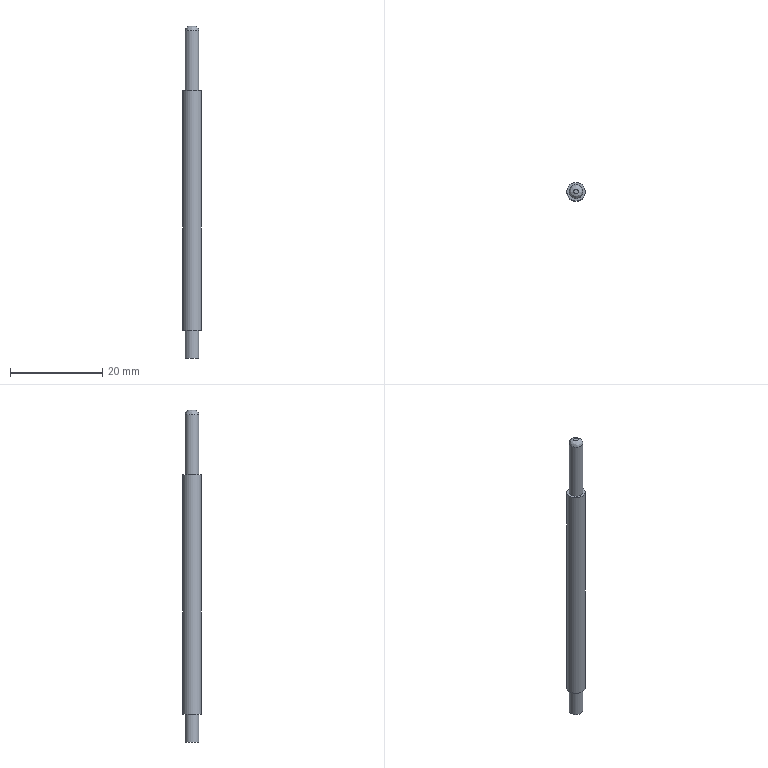Component | NX | CONN_SHAFT_1 | 1 solid | 8 faces | box 4 x 4 x 72 mm | volume 793 mm3 | plane 4 | cylinder 3 | spline 1 | commonest cylinder face diameters 3 x2 4 x1
STEP:
#1=CARTESIAN_POINT('',(0.,0.,0.));
#2=DIRECTION('',(0.,0.,1.));
#3=DIRECTION('',(1.,0.,0.));
#4=AXIS2_PLACEMENT_3D('',#1,#2,#3);
#5=CARTESIAN_POINT('',(0.004666,23.5,164.631));
#6=VERTEX_POINT('',#5);
#7=CARTESIAN_POINT('',(-0.,23.,164.631));
#8=DIRECTION('',(0.,0.,1.));
#9=DIRECTION('',(0.009333,1.,0.));
#10=AXIS2_PLACEMENT_3D('',#7,#8,#9);
#11=CIRCLE('',#10,0.5);
#12=CARTESIAN_POINT('',(-0.,23.,164.631));
#13=DIRECTION('',(0.,0.,1.));
#14=DIRECTION('',(0.009333,1.,0.));
#15=AXIS2_PLACEMENT_3D('',#12,#13,#14);
#16=PLANE('',#15);
#17=CARTESIAN_POINT('',(0.,0.));
#18=DIRECTION('',(1.,0.));
#19=AXIS2_PLACEMENT_2D('',#17,#18);
#20=CIRCLE('',#19,0.5);
#21=(GEOMETRIC_REPRESENTATION_CONTEXT(2)PARAMETRIC_REPRESENTATION_CONTEXT()REPRESENTATION_CONTEXT('',''));
#22=DEFINITIONAL_REPRESENTATION('',(#20),#21);
#23=PCURVE('',#16,#22);
#24=CARTESIAN_POINT('',(0.004666,23.5,164.631));
#25=CARTESIAN_POINT('',(-0.9953,23.509,164.631));
#26=CARTESIAN_POINT('',(-1.005,22.509,164.631));
#27=CARTESIAN_POINT('',(-0.004666,22.5,164.631));
#28=CARTESIAN_POINT('',(0.9953,22.491,164.631));
#29=CARTESIAN_POINT('',(1.005,23.491,164.631));
#30=CARTESIAN_POINT('',(0.004666,23.5,164.631));
#31=CARTESIAN_POINT('',(0.01013,24.086,164.631));
#32=CARTESIAN_POINT('',(-2.161,24.106,164.631));
#33=CARTESIAN_POINT('',(-2.182,21.935,164.631));
#34=CARTESIAN_POINT('',(-0.01013,21.914,164.631));
#35=CARTESIAN_POINT('',(2.161,21.894,164.631));
#36=CARTESIAN_POINT('',(2.182,24.065,164.631));
#37=CARTESIAN_POINT('',(0.01013,24.086,164.631));
#38=CARTESIAN_POINT('',(0.014,24.5,164.217));
#39=CARTESIAN_POINT('',(-2.986,24.528,164.217));
#40=CARTESIAN_POINT('',(-3.014,21.528,164.217));
#41=CARTESIAN_POINT('',(-0.014,21.5,164.217));
#42=CARTESIAN_POINT('',(2.986,21.472,164.217));
#43=CARTESIAN_POINT('',(3.014,24.472,164.217));
#44=CARTESIAN_POINT('',(0.014,24.5,164.217));
#45=CARTESIAN_POINT('',(0.014,24.5,163.631));
#46=CARTESIAN_POINT('',(-2.986,24.528,163.631));
#47=CARTESIAN_POINT('',(-3.014,21.528,163.631));
#48=CARTESIAN_POINT('',(-0.014,21.5,163.631));
#49=CARTESIAN_POINT('',(2.986,21.472,163.631));
#50=CARTESIAN_POINT('',(3.014,24.472,163.631));
#51=CARTESIAN_POINT('',(0.014,24.5,163.631));
#52=(BOUNDED_SURFACE()B_SPLINE_SURFACE(3,3,((#24,#25,#26,#27,#28,#29,#30),(#31,#32,#33,#34,#35,#36,#37),(#38,#39,#40,#41,#42,#43,#44),(#45,#46,#47,#48,#49,#50,#51)),.UNSPECIFIED.,.F.,.T.,.F.)B_SPLINE_SURFACE_WITH_KNOTS((4,4),(1,3,3,3,1),(0.,1.),(-0.5,0.,0.5,1.,1.5),.UNSPECIFIED.)GEOMETRIC_REPRESENTATION_ITEM()RATIONAL_B_SPLINE_SURFACE(((1.,0.3333,0.3333,1.,0.3333,0.3333,1.),(0.8047,0.2682,0.2682,0.8047,0.2682,0.2682,0.8047),(0.8047,0.2682,0.2682,0.8047,0.2682,0.2682,0.8047),(1.,0.3333,0.3333,1.,0.3333,0.3333,1.)))REPRESENTATION_ITEM('')SURFACE());
#53=CARTESIAN_POINT('',(0.,0.));
#54=CARTESIAN_POINT('',(0.,0.02352));
#55=CARTESIAN_POINT('',(0.,0.06491));
#56=CARTESIAN_POINT('',(0.,0.1146));
#57=CARTESIAN_POINT('',(0.,0.1575));
#58=CARTESIAN_POINT('',(0.,0.196));
#59=CARTESIAN_POINT('',(0.,0.2322));
#60=CARTESIAN_POINT('',(0.,0.2678));
#61=CARTESIAN_POINT('',(0.,0.304));
#62=CARTESIAN_POINT('',(0.,0.3425));
#63=CARTESIAN_POINT('',(0.,0.3856));
#64=CARTESIAN_POINT('',(0.,0.4343));
#65=CARTESIAN_POINT('',(0.,0.5));
#66=CARTESIAN_POINT('',(0.,0.5657));
#67=CARTESIAN_POINT('',(0.,0.6144));
#68=CARTESIAN_POINT('',(0.,0.6575));
#69=CARTESIAN_POINT('',(0.,0.696));
#70=CARTESIAN_POINT('',(0.,0.7322));
#71=CARTESIAN_POINT('',(0.,0.7678));
#72=CARTESIAN_POINT('',(0.,0.804));
#73=CARTESIAN_POINT('',(0.,0.8425));
#74=CARTESIAN_POINT('',(0.,0.8854));
#75=CARTESIAN_POINT('',(0.,0.9351));
#76=CARTESIAN_POINT('',(0.,0.9765));
#77=CARTESIAN_POINT('',(0.,1.));
#78=B_SPLINE_CURVE_WITH_KNOTS('',3,(#53,#54,#55,#56,#57,#58,#59,#60,#61,#62,#63,#64,#65,#66,#67,#68,#69,#70,#71,#72,#73,#74,#75,#76,#77),.UNSPECIFIED.,.F.,.F.,(4,1,1,1,1,1,1,1,1,1,1,1,1,1,1,1,1,1,1,1,1,1,4),(0.,0.2856,0.5712,0.8568,1.142,1.428,1.714,1.999,2.285,2.57,2.856,3.142,3.427,3.713,3.998,4.284,4.57,4.855,5.141,5.426,5.712,5.998,6.283),.QUASI_UNIFORM_KNOTS.);
#79=(GEOMETRIC_REPRESENTATION_CONTEXT(2)PARAMETRIC_REPRESENTATION_CONTEXT()REPRESENTATION_CONTEXT('',''));
#80=DEFINITIONAL_REPRESENTATION('',(#78),#79);
#81=PCURVE('',#52,#80);
#82=SURFACE_CURVE('',#11,(#23,#81),.PCURVE_S1.);
#83=EDGE_CURVE('',#6,#6,#82,.T.);
#84=ORIENTED_EDGE('',*,*,#83,.T.);
#85=EDGE_LOOP('',(#84));
#86=FACE_BOUND('',#85,.T.);
#87=ADVANCED_FACE('',(#86),#16,.T.);
#88=CARTESIAN_POINT('',(0.014,24.5,163.631));
#89=VERTEX_POINT('',#88);
#90=CARTESIAN_POINT('',(-0.,23.,163.631));
#91=DIRECTION('',(0.,0.,-1.));
#92=DIRECTION('',(0.009333,1.,0.));
#93=AXIS2_PLACEMENT_3D('',#90,#91,#92);
#94=CIRCLE('',#93,1.5);
#95=CARTESIAN_POINT('',(-0.,23.,150.631));
#96=DIRECTION('',(0.,0.,1.));
#97=DIRECTION('',(0.009333,1.,0.));
#98=AXIS2_PLACEMENT_3D('',#95,#96,#97);
#99=CYLINDRICAL_SURFACE('',#98,1.5);
#100=CARTESIAN_POINT('',(6.283,13.));
#101=DIRECTION('',(-1.,0.));
#102=VECTOR('',#101,1.);
#103=LINE('',#100,#102);
#104=(GEOMETRIC_REPRESENTATION_CONTEXT(2)PARAMETRIC_REPRESENTATION_CONTEXT()REPRESENTATION_CONTEXT('',''));
#105=DEFINITIONAL_REPRESENTATION('',(#103),#104);
#106=PCURVE('',#99,#105);
#107=CARTESIAN_POINT('',(1.,1.));
#108=CARTESIAN_POINT('',(1.,0.9765));
#109=CARTESIAN_POINT('',(1.,0.9351));
#110=CARTESIAN_POINT('',(1.,0.8854));
#111=CARTESIAN_POINT('',(1.,0.8425));
#112=CARTESIAN_POINT('',(1.,0.804));
#113=CARTESIAN_POINT('',(1.,0.7678));
#114=CARTESIAN_POINT('',(1.,0.7322));
#115=CARTESIAN_POINT('',(1.,0.696));
#116=CARTESIAN_POINT('',(1.,0.6575));
#117=CARTESIAN_POINT('',(1.,0.6144));
#118=CARTESIAN_POINT('',(1.,0.5657));
#119=CARTESIAN_POINT('',(1.,0.5));
#120=CARTESIAN_POINT('',(1.,0.4343));
#121=CARTESIAN_POINT('',(1.,0.3856));
#122=CARTESIAN_POINT('',(1.,0.3425));
#123=CARTESIAN_POINT('',(1.,0.304));
#124=CARTESIAN_POINT('',(1.,0.2678));
#125=CARTESIAN_POINT('',(1.,0.2322));
#126=CARTESIAN_POINT('',(1.,0.196));
#127=CARTESIAN_POINT('',(1.,0.1575));
#128=CARTESIAN_POINT('',(1.,0.1146));
#129=CARTESIAN_POINT('',(1.,0.06491));
#130=CARTESIAN_POINT('',(1.,0.02352));
#131=CARTESIAN_POINT('',(1.,0.));
#132=B_SPLINE_CURVE_WITH_KNOTS('',3,(#107,#108,#109,#110,#111,#112,#113,#114,#115,#116,#117,#118,#119,#120,#121,#122,#123,#124,#125,#126,#127,#128,#129,#130,#131),.UNSPECIFIED.,.F.,.F.,(4,1,1,1,1,1,1,1,1,1,1,1,1,1,1,1,1,1,1,1,1,1,4),(0.,0.2856,0.5712,0.8568,1.142,1.428,1.714,1.999,2.285,2.57,2.856,3.142,3.427,3.713,3.998,4.284,4.57,4.855,5.141,5.426,5.712,5.998,6.283),.QUASI_UNIFORM_KNOTS.);
#133=(GEOMETRIC_REPRESENTATION_CONTEXT(2)PARAMETRIC_REPRESENTATION_CONTEXT()REPRESENTATION_CONTEXT('',''));
#134=DEFINITIONAL_REPRESENTATION('',(#132),#133);
#135=PCURVE('',#52,#134);
#136=SURFACE_CURVE('',#94,(#106,#135),.PCURVE_S1.);
#137=EDGE_CURVE('',#89,#89,#136,.T.);
#138=ORIENTED_EDGE('',*,*,#137,.T.);
#139=CARTESIAN_POINT('',(0.014,24.5,150.631));
#140=VERTEX_POINT('',#139);
#141=CARTESIAN_POINT('',(0.014,24.5,150.631));
#142=CARTESIAN_POINT('',(0.014,24.5,163.631));
#143=B_SPLINE_CURVE_WITH_KNOTS('',1,(#141,#142),.UNSPECIFIED.,.F.,.F.,(2,2),(0.,13.),.PIECEWISE_BEZIER_KNOTS.);
#144=CARTESIAN_POINT('',(0.,0.));
#145=DIRECTION('',(0.,1.));
#146=VECTOR('',#145,1.);
#147=LINE('',#144,#146);
#148=(GEOMETRIC_REPRESENTATION_CONTEXT(2)PARAMETRIC_REPRESENTATION_CONTEXT()REPRESENTATION_CONTEXT('',''));
#149=DEFINITIONAL_REPRESENTATION('',(#147),#148);
#150=PCURVE('',#99,#149);
#151=CARTESIAN_POINT('',(6.283,0.));
#152=DIRECTION('',(0.,1.));
#153=VECTOR('',#152,1.);
#154=LINE('',#151,#153);
#155=(GEOMETRIC_REPRESENTATION_CONTEXT(2)PARAMETRIC_REPRESENTATION_CONTEXT()REPRESENTATION_CONTEXT('',''));
#156=DEFINITIONAL_REPRESENTATION('',(#154),#155);
#157=PCURVE('',#99,#156);
#158=SEAM_CURVE('',#143,(#150,#157),.PCURVE_S1.);
#159=EDGE_CURVE('',#140,#89,#158,.T.);
#160=ORIENTED_EDGE('',*,*,#159,.F.);
#161=CARTESIAN_POINT('',(-0.,23.,150.631));
#162=DIRECTION('',(0.,0.,1.));
#163=DIRECTION('',(0.009333,1.,0.));
#164=AXIS2_PLACEMENT_3D('',#161,#162,#163);
#165=CIRCLE('',#164,1.5);
#166=CARTESIAN_POINT('',(0.,0.));
#167=DIRECTION('',(1.,0.));
#168=VECTOR('',#167,1.);
#169=LINE('',#166,#168);
#170=(GEOMETRIC_REPRESENTATION_CONTEXT(2)PARAMETRIC_REPRESENTATION_CONTEXT()REPRESENTATION_CONTEXT('',''));
#171=DEFINITIONAL_REPRESENTATION('',(#169),#170);
#172=PCURVE('',#99,#171);
#173=CARTESIAN_POINT('',(-0.,23.,150.631));
#174=DIRECTION('',(0.,0.,1.));
#175=DIRECTION('',(0.009333,1.,0.));
#176=AXIS2_PLACEMENT_3D('',#173,#174,#175);
#177=PLANE('',#176);
#178=CARTESIAN_POINT('',(0.,-0.));
#179=DIRECTION('',(1.,0.));
#180=AXIS2_PLACEMENT_2D('',#178,#179);
#181=CIRCLE('',#180,1.5);
#182=(GEOMETRIC_REPRESENTATION_CONTEXT(2)PARAMETRIC_REPRESENTATION_CONTEXT()REPRESENTATION_CONTEXT('',''));
#183=DEFINITIONAL_REPRESENTATION('',(#181),#182);
#184=PCURVE('',#177,#183);
#185=SURFACE_CURVE('',#165,(#172,#184),.PCURVE_S1.);
#186=EDGE_CURVE('',#140,#140,#185,.T.);
#187=ORIENTED_EDGE('',*,*,#186,.T.);
#188=ORIENTED_EDGE('',*,*,#159,.T.);
#189=EDGE_LOOP('',(#138,#160,#187,#188));
#190=FACE_BOUND('',#189,.T.);
#191=ADVANCED_FACE('',(#190),#99,.T.);
#192=CARTESIAN_POINT('',(-0.014,21.5,98.631));
#193=VERTEX_POINT('',#192);
#194=CARTESIAN_POINT('',(-0.,23.,98.631));
#195=DIRECTION('',(0.,0.,-1.));
#196=DIRECTION('',(-0.009333,-1.,0.));
#197=AXIS2_PLACEMENT_3D('',#194,#195,#196);
#198=CIRCLE('',#197,1.5);
#199=CARTESIAN_POINT('',(-0.,23.,98.631));
#200=DIRECTION('',(0.,0.,-1.));
#201=DIRECTION('',(-0.009333,-1.,0.));
#202=AXIS2_PLACEMENT_3D('',#199,#200,#201);
#203=PLANE('',#202);
#204=CARTESIAN_POINT('',(-0.,-0.));
#205=DIRECTION('',(1.,0.));
#206=AXIS2_PLACEMENT_2D('',#204,#205);
#207=CIRCLE('',#206,1.5);
#208=(GEOMETRIC_REPRESENTATION_CONTEXT(2)PARAMETRIC_REPRESENTATION_CONTEXT()REPRESENTATION_CONTEXT('',''));
#209=DEFINITIONAL_REPRESENTATION('',(#207),#208);
#210=PCURVE('',#203,#209);
#211=CARTESIAN_POINT('',(-0.,23.,98.631));
#212=DIRECTION('',(0.,0.,-1.));
#213=DIRECTION('',(-0.009333,-1.,0.));
#214=AXIS2_PLACEMENT_3D('',#211,#212,#213);
#215=CYLINDRICAL_SURFACE('',#214,1.5);
#216=CARTESIAN_POINT('',(0.,0.));
#217=DIRECTION('',(1.,0.));
#218=VECTOR('',#217,1.);
#219=LINE('',#216,#218);
#220=(GEOMETRIC_REPRESENTATION_CONTEXT(2)PARAMETRIC_REPRESENTATION_CONTEXT()REPRESENTATION_CONTEXT('',''));
#221=DEFINITIONAL_REPRESENTATION('',(#219),#220);
#222=PCURVE('',#215,#221);
#223=SURFACE_CURVE('',#198,(#210,#222),.PCURVE_S1.);
#224=EDGE_CURVE('',#193,#193,#223,.T.);
#225=ORIENTED_EDGE('',*,*,#224,.F.);
#226=EDGE_LOOP('',(#225));
#227=FACE_BOUND('',#226,.T.);
#228=CARTESIAN_POINT('',(-0.01867,21.,98.631));
#229=VERTEX_POINT('',#228);
#230=CARTESIAN_POINT('',(-0.,23.,98.631));
#231=DIRECTION('',(0.,0.,-1.));
#232=DIRECTION('',(-0.009333,-1.,0.));
#233=AXIS2_PLACEMENT_3D('',#230,#231,#232);
#234=CIRCLE('',#233,2.);
#235=CARTESIAN_POINT('',(0.,0.));
#236=DIRECTION('',(1.,0.));
#237=AXIS2_PLACEMENT_2D('',#235,#236);
#238=CIRCLE('',#237,2.);
#239=(GEOMETRIC_REPRESENTATION_CONTEXT(2)PARAMETRIC_REPRESENTATION_CONTEXT()REPRESENTATION_CONTEXT('',''));
#240=DEFINITIONAL_REPRESENTATION('',(#238),#239);
#241=PCURVE('',#203,#240);
#242=CARTESIAN_POINT('',(-0.,23.,150.631));
#243=DIRECTION('',(0.,0.,-1.));
#244=DIRECTION('',(-0.009333,-1.,0.));
#245=AXIS2_PLACEMENT_3D('',#242,#243,#244);
#246=CYLINDRICAL_SURFACE('',#245,2.);
#247=CARTESIAN_POINT('',(0.,52.));
#248=DIRECTION('',(1.,0.));
#249=VECTOR('',#248,1.);
#250=LINE('',#247,#249);
#251=(GEOMETRIC_REPRESENTATION_CONTEXT(2)PARAMETRIC_REPRESENTATION_CONTEXT()REPRESENTATION_CONTEXT('',''));
#252=DEFINITIONAL_REPRESENTATION('',(#250),#251);
#253=PCURVE('',#246,#252);
#254=SURFACE_CURVE('',#234,(#241,#253),.PCURVE_S1.);
#255=EDGE_CURVE('',#229,#229,#254,.T.);
#256=ORIENTED_EDGE('',*,*,#255,.T.);
#257=EDGE_LOOP('',(#256));
#258=FACE_BOUND('',#257,.T.);
#259=ADVANCED_FACE('',(#227,#258),#203,.T.);
#260=ORIENTED_EDGE('',*,*,#186,.F.);
#261=EDGE_LOOP('',(#260));
#262=FACE_BOUND('',#261,.T.);
#263=CARTESIAN_POINT('',(-0.01867,21.,150.631));
#264=VERTEX_POINT('',#263);
#265=CARTESIAN_POINT('',(-0.,23.,150.631));
#266=DIRECTION('',(0.,0.,-1.));
#267=DIRECTION('',(-0.009333,-1.,0.));
#268=AXIS2_PLACEMENT_3D('',#265,#266,#267);
#269=CIRCLE('',#268,2.);
#270=CARTESIAN_POINT('',(-2.,0.));
#271=CARTESIAN_POINT('',(-2.,3.464));
#272=CARTESIAN_POINT('',(1.,1.732));
#273=CARTESIAN_POINT('',(4.,0.));
#274=CARTESIAN_POINT('',(1.,-1.732));
#275=CARTESIAN_POINT('',(-2.,-3.464));
#276=CARTESIAN_POINT('',(-2.,0.));
#277=(BOUNDED_CURVE()B_SPLINE_CURVE(2,(#270,#271,#272,#273,#274,#275,#276),.UNSPECIFIED.,.T.,.F.)B_SPLINE_CURVE_WITH_KNOTS((1,2,2,2,2,1),(-2.094,0.,2.094,4.189,6.283,8.378),.UNSPECIFIED.)CURVE()GEOMETRIC_REPRESENTATION_ITEM()RATIONAL_B_SPLINE_CURVE((1.,0.5,1.,0.5,1.,0.5,1.))REPRESENTATION_ITEM(''));
#278=(GEOMETRIC_REPRESENTATION_CONTEXT(2)PARAMETRIC_REPRESENTATION_CONTEXT()REPRESENTATION_CONTEXT('',''));
#279=DEFINITIONAL_REPRESENTATION('',(#277),#278);
#280=PCURVE('',#177,#279);
#281=CARTESIAN_POINT('',(0.,0.));
#282=DIRECTION('',(1.,0.));
#283=VECTOR('',#282,1.);
#284=LINE('',#281,#283);
#285=(GEOMETRIC_REPRESENTATION_CONTEXT(2)PARAMETRIC_REPRESENTATION_CONTEXT()REPRESENTATION_CONTEXT('',''));
#286=DEFINITIONAL_REPRESENTATION('',(#284),#285);
#287=PCURVE('',#246,#286);
#288=SURFACE_CURVE('',#269,(#280,#287),.PCURVE_S1.);
#289=EDGE_CURVE('',#264,#264,#288,.T.);
#290=ORIENTED_EDGE('',*,*,#289,.F.);
#291=EDGE_LOOP('',(#290));
#292=FACE_BOUND('',#291,.T.);
#293=ADVANCED_FACE('',(#262,#292),#177,.T.);
#294=ORIENTED_EDGE('',*,*,#255,.F.);
#295=CARTESIAN_POINT('',(-0.01867,21.,150.631));
#296=CARTESIAN_POINT('',(-0.01867,21.,98.631));
#297=B_SPLINE_CURVE_WITH_KNOTS('',1,(#295,#296),.UNSPECIFIED.,.F.,.F.,(2,2),(0.,52.),.PIECEWISE_BEZIER_KNOTS.);
#298=CARTESIAN_POINT('',(0.,0.));
#299=DIRECTION('',(0.,1.));
#300=VECTOR('',#299,1.);
#301=LINE('',#298,#300);
#302=(GEOMETRIC_REPRESENTATION_CONTEXT(2)PARAMETRIC_REPRESENTATION_CONTEXT()REPRESENTATION_CONTEXT('',''));
#303=DEFINITIONAL_REPRESENTATION('',(#301),#302);
#304=PCURVE('',#246,#303);
#305=CARTESIAN_POINT('',(6.283,0.));
#306=DIRECTION('',(0.,1.));
#307=VECTOR('',#306,1.);
#308=LINE('',#305,#307);
#309=(GEOMETRIC_REPRESENTATION_CONTEXT(2)PARAMETRIC_REPRESENTATION_CONTEXT()REPRESENTATION_CONTEXT('',''));
#310=DEFINITIONAL_REPRESENTATION('',(#308),#309);
#311=PCURVE('',#246,#310);
#312=SEAM_CURVE('',#297,(#304,#311),.PCURVE_S1.);
#313=EDGE_CURVE('',#264,#229,#312,.T.);
#314=ORIENTED_EDGE('',*,*,#313,.F.);
#315=ORIENTED_EDGE('',*,*,#289,.T.);
#316=ORIENTED_EDGE('',*,*,#313,.T.);
#317=EDGE_LOOP('',(#294,#314,#315,#316));
#318=FACE_BOUND('',#317,.T.);
#319=ADVANCED_FACE('',(#318),#246,.T.);
#320=CARTESIAN_POINT('',(-0.014,21.5,92.631));
#321=VERTEX_POINT('',#320);
#322=CARTESIAN_POINT('',(-0.,23.,92.631));
#323=DIRECTION('',(0.,0.,-1.));
#324=DIRECTION('',(-0.009333,-1.,0.));
#325=AXIS2_PLACEMENT_3D('',#322,#323,#324);
#326=CIRCLE('',#325,1.5);
#327=CARTESIAN_POINT('',(-0.,23.,92.631));
#328=DIRECTION('',(0.,0.,-1.));
#329=DIRECTION('',(-0.009333,-1.,0.));
#330=AXIS2_PLACEMENT_3D('',#327,#328,#329);
#331=PLANE('',#330);
#332=CARTESIAN_POINT('',(0.,0.));
#333=DIRECTION('',(1.,0.));
#334=AXIS2_PLACEMENT_2D('',#332,#333);
#335=CIRCLE('',#334,1.5);
#336=(GEOMETRIC_REPRESENTATION_CONTEXT(2)PARAMETRIC_REPRESENTATION_CONTEXT()REPRESENTATION_CONTEXT('',''));
#337=DEFINITIONAL_REPRESENTATION('',(#335),#336);
#338=PCURVE('',#331,#337);
#339=CARTESIAN_POINT('',(0.,6.));
#340=DIRECTION('',(1.,0.));
#341=VECTOR('',#340,1.);
#342=LINE('',#339,#341);
#343=(GEOMETRIC_REPRESENTATION_CONTEXT(2)PARAMETRIC_REPRESENTATION_CONTEXT()REPRESENTATION_CONTEXT('',''));
#344=DEFINITIONAL_REPRESENTATION('',(#342),#343);
#345=PCURVE('',#215,#344);
#346=SURFACE_CURVE('',#326,(#338,#345),.PCURVE_S1.);
#347=EDGE_CURVE('',#321,#321,#346,.T.);
#348=ORIENTED_EDGE('',*,*,#347,.T.);
#349=EDGE_LOOP('',(#348));
#350=FACE_BOUND('',#349,.T.);
#351=ADVANCED_FACE('',(#350),#331,.T.);
#352=ORIENTED_EDGE('',*,*,#347,.F.);
#353=CARTESIAN_POINT('',(-0.014,21.5,98.631));
#354=CARTESIAN_POINT('',(-0.014,21.5,92.631));
#355=B_SPLINE_CURVE_WITH_KNOTS('',1,(#353,#354),.UNSPECIFIED.,.F.,.F.,(2,2),(0.,6.),.PIECEWISE_BEZIER_KNOTS.);
#356=CARTESIAN_POINT('',(0.,0.));
#357=DIRECTION('',(0.,1.));
#358=VECTOR('',#357,1.);
#359=LINE('',#356,#358);
#360=(GEOMETRIC_REPRESENTATION_CONTEXT(2)PARAMETRIC_REPRESENTATION_CONTEXT()REPRESENTATION_CONTEXT('',''));
#361=DEFINITIONAL_REPRESENTATION('',(#359),#360);
#362=PCURVE('',#215,#361);
#363=CARTESIAN_POINT('',(6.283,0.));
#364=DIRECTION('',(0.,1.));
#365=VECTOR('',#364,1.);
#366=LINE('',#363,#365);
#367=(GEOMETRIC_REPRESENTATION_CONTEXT(2)PARAMETRIC_REPRESENTATION_CONTEXT()REPRESENTATION_CONTEXT('',''));
#368=DEFINITIONAL_REPRESENTATION('',(#366),#367);
#369=PCURVE('',#215,#368);
#370=SEAM_CURVE('',#355,(#362,#369),.PCURVE_S1.);
#371=EDGE_CURVE('',#193,#321,#370,.T.);
#372=ORIENTED_EDGE('',*,*,#371,.F.);
#373=ORIENTED_EDGE('',*,*,#224,.T.);
#374=ORIENTED_EDGE('',*,*,#371,.T.);
#375=EDGE_LOOP('',(#352,#372,#373,#374));
#376=FACE_BOUND('',#375,.T.);
#377=ADVANCED_FACE('',(#376),#215,.T.);
#378=ORIENTED_EDGE('',*,*,#83,.F.);
#379=CARTESIAN_POINT('',(0.004666,23.5,164.631));
#380=CARTESIAN_POINT('',(0.01013,24.086,164.631));
#381=CARTESIAN_POINT('',(0.014,24.5,164.217));
#382=CARTESIAN_POINT('',(0.014,24.5,163.631));
#383=(BOUNDED_CURVE()B_SPLINE_CURVE(3,(#379,#380,#381,#382),.UNSPECIFIED.,.F.,.F.)B_SPLINE_CURVE_WITH_KNOTS((4,4),(0.,1.),.PIECEWISE_BEZIER_KNOTS.)CURVE()GEOMETRIC_REPRESENTATION_ITEM()RATIONAL_B_SPLINE_CURVE((1.,0.8047,0.8047,1.))REPRESENTATION_ITEM(''));
#384=CARTESIAN_POINT('',(0.,0.));
#385=DIRECTION('',(1.,0.));
#386=VECTOR('',#385,1.);
#387=LINE('',#384,#386);
#388=(GEOMETRIC_REPRESENTATION_CONTEXT(2)PARAMETRIC_REPRESENTATION_CONTEXT()REPRESENTATION_CONTEXT('',''));
#389=DEFINITIONAL_REPRESENTATION('',(#387),#388);
#390=PCURVE('',#52,#389);
#391=CARTESIAN_POINT('',(0.,1.));
#392=DIRECTION('',(1.,0.));
#393=VECTOR('',#392,1.);
#394=LINE('',#391,#393);
#395=(GEOMETRIC_REPRESENTATION_CONTEXT(2)PARAMETRIC_REPRESENTATION_CONTEXT()REPRESENTATION_CONTEXT('',''));
#396=DEFINITIONAL_REPRESENTATION('',(#394),#395);
#397=PCURVE('',#52,#396);
#398=SEAM_CURVE('',#383,(#390,#397),.PCURVE_S1.);
#399=EDGE_CURVE('',#6,#89,#398,.T.);
#400=ORIENTED_EDGE('',*,*,#399,.T.);
#401=ORIENTED_EDGE('',*,*,#137,.F.);
#402=ORIENTED_EDGE('',*,*,#399,.F.);
#403=EDGE_LOOP('',(#378,#400,#401,#402));
#404=FACE_BOUND('',#403,.T.);
#405=ADVANCED_FACE('',(#404),#52,.T.);
#406=CLOSED_SHELL('',(#87,#191,#259,#293,#319,#351,#377,#405));
#407=MANIFOLD_SOLID_BREP('',#406);
#408=(LENGTH_UNIT()NAMED_UNIT(*)SI_UNIT(.MILLI.,.METRE.));
#409=UNCERTAINTY_MEASURE_WITH_UNIT(LENGTH_MEASURE(0.00001),#408,'','');
#410=(NAMED_UNIT(*)PLANE_ANGLE_UNIT()SI_UNIT($,.RADIAN.));
#411=(NAMED_UNIT(*)SI_UNIT($,.STERADIAN.)SOLID_ANGLE_UNIT());
#412=(GEOMETRIC_REPRESENTATION_CONTEXT(3)GLOBAL_UNCERTAINTY_ASSIGNED_CONTEXT((#409))GLOBAL_UNIT_ASSIGNED_CONTEXT((#408,#410,#411))REPRESENTATION_CONTEXT('',''));
#413=ADVANCED_BREP_SHAPE_REPRESENTATION('',(#4,#407),#412);